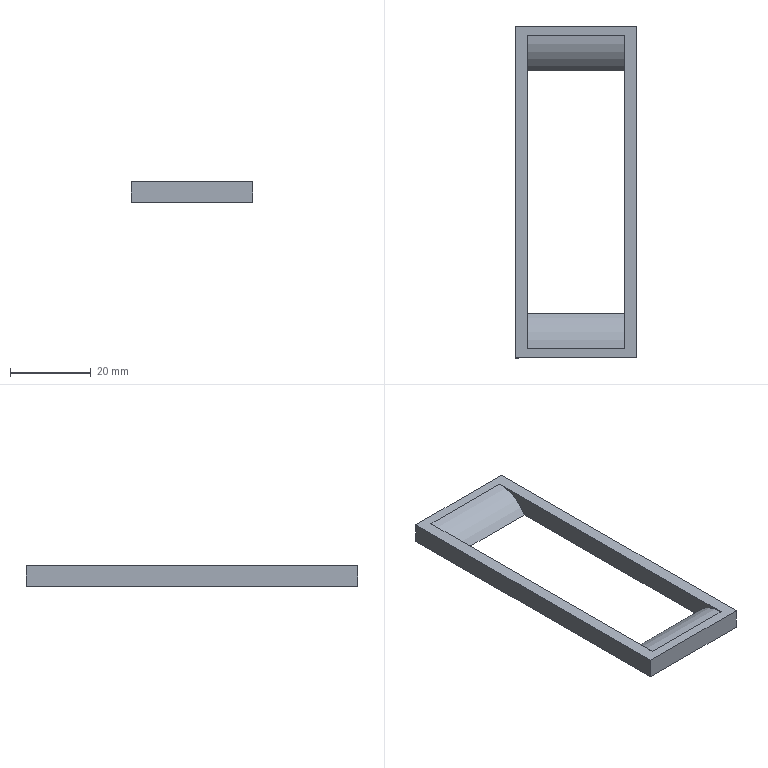Component | SolidWorks | 1UnitDrawer-1_DrawerPanelLabelFrame-1 | 1 solid | 16 faces | box 30 x 82 x 5 mm | volume 4407 mm3 | plane 10 | cylinder 6 | commonest cylinder face diameters 5.3 x4 20 x2
STEP:
#1=COLOUR_RGB('',0.7922,0.8196,0.9333);
#2=FILL_AREA_STYLE_COLOUR('',#1);
#3=FILL_AREA_STYLE('',(#2));
#4=SURFACE_STYLE_FILL_AREA(#3);
#5=SURFACE_SIDE_STYLE('',(#4));
#6=SURFACE_STYLE_USAGE(.BOTH.,#5);
#7=PRESENTATION_STYLE_ASSIGNMENT((#6));
#8=CARTESIAN_POINT('',(-72.576,-26.842,16.614));
#9=VERTEX_POINT('',#8);
#10=CARTESIAN_POINT('',(-72.576,-27.051,16.614));
#11=VERTEX_POINT('',#10);
#12=CARTESIAN_POINT('',(-72.576,-26.947,16.614));
#13=DIRECTION('',(0.,-0.,-1.));
#14=DIRECTION('',(0.,-1.,0.));
#15=AXIS2_PLACEMENT_3D('',#12,#13,#14);
#16=CIRCLE('',#15,0.1043);
#17=EDGE_CURVE('',#9,#11,#16,.T.);
#18=ORIENTED_EDGE('',*,*,#17,.F.);
#19=CARTESIAN_POINT('',(-72.576,-26.842,16.535));
#20=VERTEX_POINT('',#19);
#21=CARTESIAN_POINT('',(-72.576,-26.842,16.614));
#22=DIRECTION('',(0.,-0.,-1.));
#23=VECTOR('',#22,39.37);
#24=LINE('',#21,#23);
#25=EDGE_CURVE('',#9,#20,#24,.T.);
#26=ORIENTED_EDGE('',*,*,#25,.T.);
#27=CARTESIAN_POINT('',(-72.576,-27.051,16.535));
#28=VERTEX_POINT('',#27);
#29=CARTESIAN_POINT('',(-72.576,-26.947,16.535));
#30=DIRECTION('',(0.,-0.,-1.));
#31=DIRECTION('',(0.,-1.,0.));
#32=AXIS2_PLACEMENT_3D('',#29,#30,#31);
#33=CIRCLE('',#32,0.1043);
#34=EDGE_CURVE('',#20,#28,#33,.T.);
#35=ORIENTED_EDGE('',*,*,#34,.T.);
#36=CARTESIAN_POINT('',(-72.576,-27.051,16.614));
#37=DIRECTION('',(0.,-0.,-1.));
#38=VECTOR('',#37,39.37);
#39=LINE('',#36,#38);
#40=EDGE_CURVE('',#11,#28,#39,.T.);
#41=ORIENTED_EDGE('',*,*,#40,.F.);
#42=EDGE_LOOP('',(#18,#26,#35,#41));
#43=FACE_OUTER_BOUND('',#42,.T.);
#44=CARTESIAN_POINT('',(-72.576,-26.947,16.614));
#45=DIRECTION('',(0.,-0.,-1.));
#46=DIRECTION('',(0.,-1.,0.));
#47=AXIS2_PLACEMENT_3D('',#44,#45,#46);
#48=CYLINDRICAL_SURFACE('',#47,0.1043);
#49=ADVANCED_FACE('',(#43),#48,.F.);
#50=CARTESIAN_POINT('',(-72.576,-23.889,16.614));
#51=VERTEX_POINT('',#50);
#52=CARTESIAN_POINT('',(-72.576,-24.098,16.614));
#53=VERTEX_POINT('',#52);
#54=CARTESIAN_POINT('',(-72.576,-23.994,16.614));
#55=DIRECTION('',(0.,-0.,-1.));
#56=DIRECTION('',(0.,-1.,0.));
#57=AXIS2_PLACEMENT_3D('',#54,#55,#56);
#58=CIRCLE('',#57,0.1043);
#59=EDGE_CURVE('',#51,#53,#58,.T.);
#60=ORIENTED_EDGE('',*,*,#59,.F.);
#61=CARTESIAN_POINT('',(-72.576,-23.889,16.535));
#62=VERTEX_POINT('',#61);
#63=CARTESIAN_POINT('',(-72.576,-23.889,16.614));
#64=DIRECTION('',(0.,-0.,-1.));
#65=VECTOR('',#64,39.37);
#66=LINE('',#63,#65);
#67=EDGE_CURVE('',#51,#62,#66,.T.);
#68=ORIENTED_EDGE('',*,*,#67,.T.);
#69=CARTESIAN_POINT('',(-72.576,-24.098,16.535));
#70=VERTEX_POINT('',#69);
#71=CARTESIAN_POINT('',(-72.576,-23.994,16.535));
#72=DIRECTION('',(0.,-0.,-1.));
#73=DIRECTION('',(0.,-1.,0.));
#74=AXIS2_PLACEMENT_3D('',#71,#72,#73);
#75=CIRCLE('',#74,0.1043);
#76=EDGE_CURVE('',#62,#70,#75,.T.);
#77=ORIENTED_EDGE('',*,*,#76,.T.);
#78=CARTESIAN_POINT('',(-72.576,-24.098,16.614));
#79=DIRECTION('',(0.,-0.,-1.));
#80=VECTOR('',#79,39.37);
#81=LINE('',#78,#80);
#82=EDGE_CURVE('',#53,#70,#81,.T.);
#83=ORIENTED_EDGE('',*,*,#82,.F.);
#84=EDGE_LOOP('',(#60,#68,#77,#83));
#85=FACE_OUTER_BOUND('',#84,.T.);
#86=CARTESIAN_POINT('',(-72.576,-23.994,16.614));
#87=DIRECTION('',(0.,-0.,-1.));
#88=DIRECTION('',(0.,-1.,0.));
#89=AXIS2_PLACEMENT_3D('',#86,#87,#88);
#90=CYLINDRICAL_SURFACE('',#89,0.1043);
#91=ADVANCED_FACE('',(#85),#90,.F.);
#92=CARTESIAN_POINT('',(-71.985,-23.856,16.732));
#93=VERTEX_POINT('',#92);
#94=CARTESIAN_POINT('',(-73.167,-23.856,16.732));
#95=VERTEX_POINT('',#94);
#96=CARTESIAN_POINT('',(-71.985,-23.856,16.732));
#97=DIRECTION('',(-1.,-0.,-0.));
#98=VECTOR('',#97,39.37);
#99=LINE('',#96,#98);
#100=EDGE_CURVE('',#93,#95,#99,.T.);
#101=ORIENTED_EDGE('',*,*,#100,.T.);
#102=CARTESIAN_POINT('',(-73.167,-27.084,16.732));
#103=VERTEX_POINT('',#102);
#104=CARTESIAN_POINT('',(-73.167,-27.084,16.732));
#105=DIRECTION('',(0.,-1.,0.));
#106=VECTOR('',#105,39.37);
#107=LINE('',#104,#106);
#108=EDGE_CURVE('',#95,#103,#107,.T.);
#109=ORIENTED_EDGE('',*,*,#108,.T.);
#110=CARTESIAN_POINT('',(-71.985,-27.084,16.732));
#111=VERTEX_POINT('',#110);
#112=CARTESIAN_POINT('',(-71.985,-27.084,16.732));
#113=DIRECTION('',(1.,0.,0.));
#114=VECTOR('',#113,39.37);
#115=LINE('',#112,#114);
#116=EDGE_CURVE('',#103,#111,#115,.T.);
#117=ORIENTED_EDGE('',*,*,#116,.T.);
#118=CARTESIAN_POINT('',(-71.985,-27.084,16.732));
#119=DIRECTION('',(-0.,1.,-0.));
#120=VECTOR('',#119,39.37);
#121=LINE('',#118,#120);
#122=EDGE_CURVE('',#111,#93,#121,.T.);
#123=ORIENTED_EDGE('',*,*,#122,.T.);
#124=EDGE_LOOP('',(#101,#109,#117,#123));
#125=FACE_OUTER_BOUND('',#124,.T.);
#126=CARTESIAN_POINT('',(-73.048,-23.948,16.732));
#127=VERTEX_POINT('',#126);
#128=CARTESIAN_POINT('',(-73.048,-26.992,16.732));
#129=VERTEX_POINT('',#128);
#130=CARTESIAN_POINT('',(-73.048,-26.651,16.732));
#131=DIRECTION('',(0.,-1.,0.));
#132=VECTOR('',#131,39.37);
#133=LINE('',#130,#132);
#134=EDGE_CURVE('',#127,#129,#133,.T.);
#135=ORIENTED_EDGE('',*,*,#134,.F.);
#136=CARTESIAN_POINT('',(-72.104,-23.948,16.732));
#137=VERTEX_POINT('',#136);
#138=CARTESIAN_POINT('',(-73.167,-23.948,16.732));
#139=DIRECTION('',(1.,0.,0.));
#140=VECTOR('',#139,39.37);
#141=LINE('',#138,#140);
#142=EDGE_CURVE('',#127,#137,#141,.T.);
#143=ORIENTED_EDGE('',*,*,#142,.T.);
#144=CARTESIAN_POINT('',(-72.104,-26.992,16.732));
#145=VERTEX_POINT('',#144);
#146=CARTESIAN_POINT('',(-72.104,-26.651,16.732));
#147=DIRECTION('',(-0.,1.,-0.));
#148=VECTOR('',#147,39.37);
#149=LINE('',#146,#148);
#150=EDGE_CURVE('',#145,#137,#149,.T.);
#151=ORIENTED_EDGE('',*,*,#150,.F.);
#152=CARTESIAN_POINT('',(-73.167,-26.992,16.732));
#153=DIRECTION('',(-1.,-0.,-0.));
#154=VECTOR('',#153,39.37);
#155=LINE('',#152,#154);
#156=EDGE_CURVE('',#145,#129,#155,.T.);
#157=ORIENTED_EDGE('',*,*,#156,.T.);
#158=EDGE_LOOP('',(#135,#143,#151,#157));
#159=FACE_BOUND('',#158,.T.);
#160=CARTESIAN_POINT('',(-73.167,-23.856,16.732));
#161=DIRECTION('',(0.,-0.,-1.));
#162=DIRECTION('',(0.,-1.,0.));
#163=AXIS2_PLACEMENT_3D('',#160,#161,#162);
#164=PLANE('',#163);
#165=ADVANCED_FACE('',(#125,#159),#164,.F.);
#166=CARTESIAN_POINT('',(-72.576,-26.947,16.535));
#167=DIRECTION('',(0.,-0.,-1.));
#168=DIRECTION('',(0.,-1.,0.));
#169=AXIS2_PLACEMENT_3D('',#166,#167,#168);
#170=CIRCLE('',#169,0.1043);
#171=EDGE_CURVE('',#28,#20,#170,.T.);
#172=ORIENTED_EDGE('',*,*,#171,.F.);
#173=ORIENTED_EDGE('',*,*,#34,.F.);
#174=EDGE_LOOP('',(#172,#173));
#175=FACE_BOUND('',#174,.T.);
#176=CARTESIAN_POINT('',(-72.576,-23.994,16.535));
#177=DIRECTION('',(0.,-0.,-1.));
#178=DIRECTION('',(0.,-1.,0.));
#179=AXIS2_PLACEMENT_3D('',#176,#177,#178);
#180=CIRCLE('',#179,0.1043);
#181=EDGE_CURVE('',#70,#62,#180,.T.);
#182=ORIENTED_EDGE('',*,*,#181,.F.);
#183=ORIENTED_EDGE('',*,*,#76,.F.);
#184=EDGE_LOOP('',(#182,#183));
#185=FACE_BOUND('',#184,.T.);
#186=CARTESIAN_POINT('',(-71.985,-23.856,16.535));
#187=VERTEX_POINT('',#186);
#188=CARTESIAN_POINT('',(-73.167,-23.856,16.535));
#189=VERTEX_POINT('',#188);
#190=CARTESIAN_POINT('',(-71.985,-23.856,16.535));
#191=DIRECTION('',(-1.,-0.,-0.));
#192=VECTOR('',#191,39.37);
#193=LINE('',#190,#192);
#194=EDGE_CURVE('',#187,#189,#193,.T.);
#195=ORIENTED_EDGE('',*,*,#194,.F.);
#196=CARTESIAN_POINT('',(-71.985,-27.084,16.535));
#197=VERTEX_POINT('',#196);
#198=CARTESIAN_POINT('',(-71.985,-27.084,16.535));
#199=DIRECTION('',(-0.,1.,-0.));
#200=VECTOR('',#199,39.37);
#201=LINE('',#198,#200);
#202=EDGE_CURVE('',#197,#187,#201,.T.);
#203=ORIENTED_EDGE('',*,*,#202,.F.);
#204=CARTESIAN_POINT('',(-73.167,-27.084,16.535));
#205=VERTEX_POINT('',#204);
#206=CARTESIAN_POINT('',(-71.985,-27.084,16.535));
#207=DIRECTION('',(1.,0.,0.));
#208=VECTOR('',#207,39.37);
#209=LINE('',#206,#208);
#210=EDGE_CURVE('',#205,#197,#209,.T.);
#211=ORIENTED_EDGE('',*,*,#210,.F.);
#212=CARTESIAN_POINT('',(-73.167,-27.084,16.535));
#213=DIRECTION('',(0.,-1.,0.));
#214=VECTOR('',#213,39.37);
#215=LINE('',#212,#214);
#216=EDGE_CURVE('',#189,#205,#215,.T.);
#217=ORIENTED_EDGE('',*,*,#216,.F.);
#218=EDGE_LOOP('',(#195,#203,#211,#217));
#219=FACE_OUTER_BOUND('',#218,.T.);
#220=CARTESIAN_POINT('',(-72.104,-26.651,16.535));
#221=VERTEX_POINT('',#220);
#222=CARTESIAN_POINT('',(-72.104,-24.289,16.535));
#223=VERTEX_POINT('',#222);
#224=CARTESIAN_POINT('',(-72.104,-26.651,16.535));
#225=DIRECTION('',(-0.,1.,-0.));
#226=VECTOR('',#225,39.37);
#227=LINE('',#224,#226);
#228=EDGE_CURVE('',#221,#223,#227,.T.);
#229=ORIENTED_EDGE('',*,*,#228,.T.);
#230=CARTESIAN_POINT('',(-73.048,-24.289,16.535));
#231=VERTEX_POINT('',#230);
#232=CARTESIAN_POINT('',(-72.104,-24.289,16.535));
#233=DIRECTION('',(-1.,-0.,-0.));
#234=VECTOR('',#233,39.37);
#235=LINE('',#232,#234);
#236=EDGE_CURVE('',#223,#231,#235,.T.);
#237=ORIENTED_EDGE('',*,*,#236,.T.);
#238=CARTESIAN_POINT('',(-73.048,-26.651,16.535));
#239=VERTEX_POINT('',#238);
#240=CARTESIAN_POINT('',(-73.048,-26.651,16.535));
#241=DIRECTION('',(0.,-1.,0.));
#242=VECTOR('',#241,39.37);
#243=LINE('',#240,#242);
#244=EDGE_CURVE('',#231,#239,#243,.T.);
#245=ORIENTED_EDGE('',*,*,#244,.T.);
#246=CARTESIAN_POINT('',(-72.104,-26.651,16.535));
#247=DIRECTION('',(1.,0.,0.));
#248=VECTOR('',#247,39.37);
#249=LINE('',#246,#248);
#250=EDGE_CURVE('',#239,#221,#249,.T.);
#251=ORIENTED_EDGE('',*,*,#250,.T.);
#252=EDGE_LOOP('',(#229,#237,#245,#251));
#253=FACE_BOUND('',#252,.T.);
#254=CARTESIAN_POINT('',(-73.167,-23.856,16.535));
#255=DIRECTION('',(0.,-0.,-1.));
#256=DIRECTION('',(0.,-1.,0.));
#257=AXIS2_PLACEMENT_3D('',#254,#255,#256);
#258=PLANE('',#257);
#259=ADVANCED_FACE('',(#175,#185,#219,#253),#258,.T.);
#260=ORIENTED_EDGE('',*,*,#194,.T.);
#261=CARTESIAN_POINT('',(-73.167,-23.856,16.732));
#262=DIRECTION('',(0.,-0.,-1.));
#263=VECTOR('',#262,39.37);
#264=LINE('',#261,#263);
#265=EDGE_CURVE('',#95,#189,#264,.T.);
#266=ORIENTED_EDGE('',*,*,#265,.F.);
#267=ORIENTED_EDGE('',*,*,#100,.F.);
#268=CARTESIAN_POINT('',(-71.985,-23.856,16.732));
#269=DIRECTION('',(0.,-0.,-1.));
#270=VECTOR('',#269,39.37);
#271=LINE('',#268,#270);
#272=EDGE_CURVE('',#93,#187,#271,.T.);
#273=ORIENTED_EDGE('',*,*,#272,.T.);
#274=EDGE_LOOP('',(#260,#266,#267,#273));
#275=FACE_OUTER_BOUND('',#274,.T.);
#276=CARTESIAN_POINT('',(-71.985,-23.856,16.732));
#277=DIRECTION('',(0.,-1.,0.));
#278=DIRECTION('',(-0.,0.,1.));
#279=AXIS2_PLACEMENT_3D('',#276,#277,#278);
#280=PLANE('',#279);
#281=ADVANCED_FACE('',(#275),#280,.F.);
#282=ORIENTED_EDGE('',*,*,#216,.T.);
#283=CARTESIAN_POINT('',(-73.167,-27.084,16.732));
#284=DIRECTION('',(0.,-0.,-1.));
#285=VECTOR('',#284,39.37);
#286=LINE('',#283,#285);
#287=EDGE_CURVE('',#103,#205,#286,.T.);
#288=ORIENTED_EDGE('',*,*,#287,.F.);
#289=ORIENTED_EDGE('',*,*,#108,.F.);
#290=ORIENTED_EDGE('',*,*,#265,.T.);
#291=EDGE_LOOP('',(#282,#288,#289,#290));
#292=FACE_OUTER_BOUND('',#291,.T.);
#293=CARTESIAN_POINT('',(-73.167,-27.084,16.732));
#294=DIRECTION('',(1.,0.,0.));
#295=DIRECTION('',(0.,-0.,-1.));
#296=AXIS2_PLACEMENT_3D('',#293,#294,#295);
#297=PLANE('',#296);
#298=ADVANCED_FACE('',(#292),#297,.F.);
#299=ORIENTED_EDGE('',*,*,#210,.T.);
#300=CARTESIAN_POINT('',(-71.985,-27.084,16.732));
#301=DIRECTION('',(0.,-0.,-1.));
#302=VECTOR('',#301,39.37);
#303=LINE('',#300,#302);
#304=EDGE_CURVE('',#111,#197,#303,.T.);
#305=ORIENTED_EDGE('',*,*,#304,.F.);
#306=ORIENTED_EDGE('',*,*,#116,.F.);
#307=ORIENTED_EDGE('',*,*,#287,.T.);
#308=EDGE_LOOP('',(#299,#305,#306,#307));
#309=FACE_OUTER_BOUND('',#308,.T.);
#310=CARTESIAN_POINT('',(-71.985,-27.084,16.732));
#311=DIRECTION('',(-0.,1.,-0.));
#312=DIRECTION('',(0.,-0.,-1.));
#313=AXIS2_PLACEMENT_3D('',#310,#311,#312);
#314=PLANE('',#313);
#315=ADVANCED_FACE('',(#309),#314,.F.);
#316=ORIENTED_EDGE('',*,*,#202,.T.);
#317=ORIENTED_EDGE('',*,*,#272,.F.);
#318=ORIENTED_EDGE('',*,*,#122,.F.);
#319=ORIENTED_EDGE('',*,*,#304,.T.);
#320=EDGE_LOOP('',(#316,#317,#318,#319));
#321=FACE_OUTER_BOUND('',#320,.T.);
#322=CARTESIAN_POINT('',(-71.985,-27.084,16.732));
#323=DIRECTION('',(-1.,-0.,-0.));
#324=DIRECTION('',(-0.,0.,1.));
#325=AXIS2_PLACEMENT_3D('',#322,#323,#324);
#326=PLANE('',#325);
#327=ADVANCED_FACE('',(#321),#326,.F.);
#328=ORIENTED_EDGE('',*,*,#244,.F.);
#329=CARTESIAN_POINT('',(-73.048,-23.948,16.339));
#330=DIRECTION('',(-1.,-0.,-0.));
#331=DIRECTION('',(0.,-0.,-1.));
#332=AXIS2_PLACEMENT_3D('',#329,#330,#331);
#333=CIRCLE('',#332,0.3937);
#334=EDGE_CURVE('',#231,#127,#333,.T.);
#335=ORIENTED_EDGE('',*,*,#334,.T.);
#336=ORIENTED_EDGE('',*,*,#134,.T.);
#337=CARTESIAN_POINT('',(-73.048,-26.992,16.339));
#338=DIRECTION('',(-1.,-0.,-0.));
#339=DIRECTION('',(0.,-0.,-1.));
#340=AXIS2_PLACEMENT_3D('',#337,#338,#339);
#341=CIRCLE('',#340,0.3937);
#342=EDGE_CURVE('',#129,#239,#341,.T.);
#343=ORIENTED_EDGE('',*,*,#342,.T.);
#344=EDGE_LOOP('',(#328,#335,#336,#343));
#345=FACE_OUTER_BOUND('',#344,.T.);
#346=CARTESIAN_POINT('',(-73.048,-26.651,16.732));
#347=DIRECTION('',(1.,0.,0.));
#348=DIRECTION('',(0.,-0.,-1.));
#349=AXIS2_PLACEMENT_3D('',#346,#347,#348);
#350=PLANE('',#349);
#351=ADVANCED_FACE('',(#345),#350,.T.);
#352=ORIENTED_EDGE('',*,*,#228,.F.);
#353=CARTESIAN_POINT('',(-72.104,-26.992,16.339));
#354=DIRECTION('',(1.,0.,0.));
#355=DIRECTION('',(0.,0.,1.));
#356=AXIS2_PLACEMENT_3D('',#353,#354,#355);
#357=CIRCLE('',#356,0.3937);
#358=EDGE_CURVE('',#221,#145,#357,.T.);
#359=ORIENTED_EDGE('',*,*,#358,.T.);
#360=ORIENTED_EDGE('',*,*,#150,.T.);
#361=CARTESIAN_POINT('',(-72.104,-23.948,16.339));
#362=DIRECTION('',(1.,0.,0.));
#363=DIRECTION('',(0.,0.,1.));
#364=AXIS2_PLACEMENT_3D('',#361,#362,#363);
#365=CIRCLE('',#364,0.3937);
#366=EDGE_CURVE('',#137,#223,#365,.T.);
#367=ORIENTED_EDGE('',*,*,#366,.T.);
#368=EDGE_LOOP('',(#352,#359,#360,#367));
#369=FACE_OUTER_BOUND('',#368,.T.);
#370=CARTESIAN_POINT('',(-72.104,-26.651,16.732));
#371=DIRECTION('',(-1.,-0.,-0.));
#372=DIRECTION('',(-0.,0.,1.));
#373=AXIS2_PLACEMENT_3D('',#370,#371,#372);
#374=PLANE('',#373);
#375=ADVANCED_FACE('',(#369),#374,.T.);
#376=ORIENTED_EDGE('',*,*,#366,.F.);
#377=ORIENTED_EDGE('',*,*,#142,.F.);
#378=ORIENTED_EDGE('',*,*,#334,.F.);
#379=ORIENTED_EDGE('',*,*,#236,.F.);
#380=EDGE_LOOP('',(#376,#377,#378,#379));
#381=FACE_OUTER_BOUND('',#380,.T.);
#382=CARTESIAN_POINT('',(-72.104,-23.948,16.339));
#383=DIRECTION('',(1.,0.,0.));
#384=DIRECTION('',(0.,-0.,-1.));
#385=AXIS2_PLACEMENT_3D('',#382,#383,#384);
#386=CYLINDRICAL_SURFACE('',#385,0.3937);
#387=ADVANCED_FACE('',(#381),#386,.T.);
#388=ORIENTED_EDGE('',*,*,#342,.F.);
#389=ORIENTED_EDGE('',*,*,#156,.F.);
#390=ORIENTED_EDGE('',*,*,#358,.F.);
#391=ORIENTED_EDGE('',*,*,#250,.F.);
#392=EDGE_LOOP('',(#388,#389,#390,#391));
#393=FACE_OUTER_BOUND('',#392,.T.);
#394=CARTESIAN_POINT('',(-72.104,-26.992,16.339));
#395=DIRECTION('',(-1.,-0.,-0.));
#396=DIRECTION('',(0.,0.,1.));
#397=AXIS2_PLACEMENT_3D('',#394,#395,#396);
#398=CYLINDRICAL_SURFACE('',#397,0.3937);
#399=ADVANCED_FACE('',(#393),#398,.T.);
#400=ORIENTED_EDGE('',*,*,#67,.F.);
#401=CARTESIAN_POINT('',(-72.576,-23.994,16.614));
#402=DIRECTION('',(0.,-0.,-1.));
#403=DIRECTION('',(0.,-1.,0.));
#404=AXIS2_PLACEMENT_3D('',#401,#402,#403);
#405=CIRCLE('',#404,0.1043);
#406=EDGE_CURVE('',#53,#51,#405,.T.);
#407=ORIENTED_EDGE('',*,*,#406,.F.);
#408=ORIENTED_EDGE('',*,*,#82,.T.);
#409=ORIENTED_EDGE('',*,*,#181,.T.);
#410=EDGE_LOOP('',(#400,#407,#408,#409));
#411=FACE_OUTER_BOUND('',#410,.T.);
#412=CARTESIAN_POINT('',(-72.576,-23.994,16.614));
#413=DIRECTION('',(0.,-0.,-1.));
#414=DIRECTION('',(0.,-1.,0.));
#415=AXIS2_PLACEMENT_3D('',#412,#413,#414);
#416=CYLINDRICAL_SURFACE('',#415,0.1043);
#417=ADVANCED_FACE('',(#411),#416,.F.);
#418=ORIENTED_EDGE('',*,*,#406,.T.);
#419=ORIENTED_EDGE('',*,*,#59,.T.);
#420=EDGE_LOOP('',(#418,#419));
#421=FACE_OUTER_BOUND('',#420,.T.);
#422=CARTESIAN_POINT('',(-72.576,-23.994,16.614));
#423=DIRECTION('',(0.,-0.,-1.));
#424=DIRECTION('',(0.,-1.,0.));
#425=AXIS2_PLACEMENT_3D('',#422,#423,#424);
#426=PLANE('',#425);
#427=ADVANCED_FACE('',(#421),#426,.T.);
#428=ORIENTED_EDGE('',*,*,#25,.F.);
#429=CARTESIAN_POINT('',(-72.576,-26.947,16.614));
#430=DIRECTION('',(0.,-0.,-1.));
#431=DIRECTION('',(0.,-1.,0.));
#432=AXIS2_PLACEMENT_3D('',#429,#430,#431);
#433=CIRCLE('',#432,0.1043);
#434=EDGE_CURVE('',#11,#9,#433,.T.);
#435=ORIENTED_EDGE('',*,*,#434,.F.);
#436=ORIENTED_EDGE('',*,*,#40,.T.);
#437=ORIENTED_EDGE('',*,*,#171,.T.);
#438=EDGE_LOOP('',(#428,#435,#436,#437));
#439=FACE_OUTER_BOUND('',#438,.T.);
#440=CARTESIAN_POINT('',(-72.576,-26.947,16.614));
#441=DIRECTION('',(0.,-0.,-1.));
#442=DIRECTION('',(0.,-1.,0.));
#443=AXIS2_PLACEMENT_3D('',#440,#441,#442);
#444=CYLINDRICAL_SURFACE('',#443,0.1043);
#445=ADVANCED_FACE('',(#439),#444,.F.);
#446=ORIENTED_EDGE('',*,*,#434,.T.);
#447=ORIENTED_EDGE('',*,*,#17,.T.);
#448=EDGE_LOOP('',(#446,#447));
#449=FACE_OUTER_BOUND('',#448,.T.);
#450=CARTESIAN_POINT('',(-72.576,-26.947,16.614));
#451=DIRECTION('',(0.,-0.,-1.));
#452=DIRECTION('',(0.,-1.,0.));
#453=AXIS2_PLACEMENT_3D('',#450,#451,#452);
#454=PLANE('',#453);
#455=ADVANCED_FACE('',(#449),#454,.T.);
#456=CLOSED_SHELL('',(#49,#91,#165,#259,#281,#298,#315,#327,#351,#375,#387,#399,#417,#427,#445,#455));
#457=MANIFOLD_SOLID_BREP('',#456);
#458=STYLED_ITEM('',(#7),#457);
#459=(LENGTH_UNIT()NAMED_UNIT(*)SI_UNIT($,.METRE.));
#460=LENGTH_MEASURE_WITH_UNIT(LENGTH_MEASURE(0.0254),#459);
#461=DIMENSIONAL_EXPONENTS(1.,0.,0.,0.,0.,0.,0.);
#462=(CONVERSION_BASED_UNIT('',#460)LENGTH_UNIT()NAMED_UNIT(#461));
#463=UNCERTAINTY_MEASURE_WITH_UNIT(LENGTH_MEASURE(0.00001),#462,'','');
#464=(NAMED_UNIT(*)PLANE_ANGLE_UNIT()SI_UNIT($,.RADIAN.));
#465=(NAMED_UNIT(*)SI_UNIT($,.STERADIAN.)SOLID_ANGLE_UNIT());
#466=(GEOMETRIC_REPRESENTATION_CONTEXT(3)GLOBAL_UNCERTAINTY_ASSIGNED_CONTEXT((#463))GLOBAL_UNIT_ASSIGNED_CONTEXT((#462,#464,#465))REPRESENTATION_CONTEXT('',''));
#467=MECHANICAL_DESIGN_GEOMETRIC_PRESENTATION_REPRESENTATION('',(#458),#466);
#468=CARTESIAN_POINT('',(0.,0.,0.));
#469=DIRECTION('',(0.,0.,1.));
#470=DIRECTION('',(1.,0.,0.));
#471=AXIS2_PLACEMENT_3D('',#468,#469,#470);
#472=(LENGTH_UNIT()NAMED_UNIT(*)SI_UNIT($,.METRE.));
#473=LENGTH_MEASURE_WITH_UNIT(LENGTH_MEASURE(0.0254),#472);
#474=DIMENSIONAL_EXPONENTS(1.,0.,0.,0.,0.,0.,0.);
#475=(CONVERSION_BASED_UNIT('',#473)LENGTH_UNIT()NAMED_UNIT(#474));
#476=UNCERTAINTY_MEASURE_WITH_UNIT(LENGTH_MEASURE(0.00001),#475,'','');
#477=(NAMED_UNIT(*)PLANE_ANGLE_UNIT()SI_UNIT($,.RADIAN.));
#478=(NAMED_UNIT(*)SI_UNIT($,.STERADIAN.)SOLID_ANGLE_UNIT());
#479=(GEOMETRIC_REPRESENTATION_CONTEXT(3)GLOBAL_UNCERTAINTY_ASSIGNED_CONTEXT((#476))GLOBAL_UNIT_ASSIGNED_CONTEXT((#475,#477,#478))REPRESENTATION_CONTEXT('',''));
#480=ADVANCED_BREP_SHAPE_REPRESENTATION('',(#457,#471),#479);
#481=PRESENTATION_LAYER_ASSIGNMENT('','',(#458));